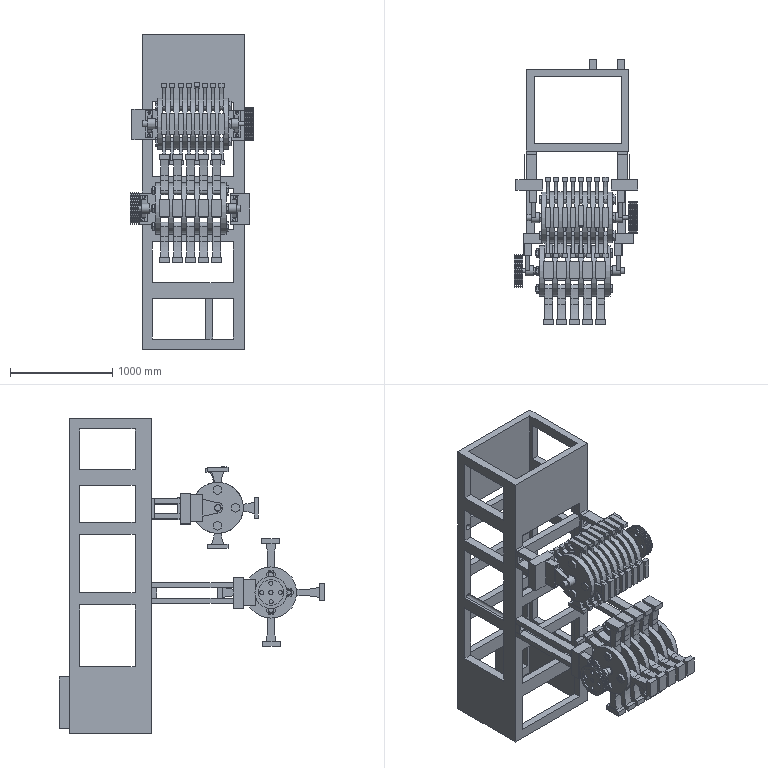Assembly | NX | mm | 108 component files | 114 solids | 1657 faces | box 1205 x 2593.88 x 3074.18 mm | volume 688918586 mm3 | plane 1034 | cylinder 559 | spline 32 | cone 32 | commonest cylinder face diameters 50 x213 1526.456 x80 580.798 x64 80 x60 60 x20 30 x16 500 x15 120 x13
Bill of materials:
unnamed part 1 | 11 |  | Thin flat circular disc with a central round bore that has a single keyway notch, and four smaller through-holes spaced evenly on a bolt circle.
unnamed part 2 | 4 |  | Rectangular mounting block with two through-holes near its ends, plus a tapered web arm that extends sideways to a cylindrical boss with a through-bore.
unnamed part 3 | 32 |  | Flat T-shaped plate: a rectangular bar head with an arm whose sides curve inward, ending in a rounded eye with a round through-hole.
unnamed part 4 | 8 |  | Hexagonal nut with a large central bore showing internal helical thread geometry; its height is small compared with its width across flats.
unnamed part 5 | 2 |  | Long open rectangular frame: two parallel bars joined by an end wall, attached to a wider rectangular end block that has two small through-holes.
unnamed part 6 | 2 |  | Long, slender, flat bar with rounded (semicircular) ends.
unnamed part 7 | 20 |  | T-shaped plate: a rectangular head block with a long arm whose sides curve slightly inward, ending in a rounded eye with a round through-hole.
unnamed part 8 | 2 |  | Multi-groove disc (pulley-like) with V-section grooves around its rim, a central bore with a keyway notch, four larger holes spaced evenly around it, and a shallow recess on the face.
unnamed part 9 | 2 |  | Stepped cylindrical shaft: a large central body with several smaller-diameter stepped sections at each end.
unnamed part 10 | 2 |  | Short open rectangular frame attached to a wide rectangular block that has two small holes on its face; the far end wall of the frame has a round hole.
unnamed part 11 | 2 |  | Thin flat circular disc with a plain central round hole and four smaller through-holes spaced evenly on a bolt circle.
unnamed part 12 | 8 |  | Long bolt-like part: a hexagonal head on a long cylindrical shank, with thread-like grooves on a short section at the far end.
unnamed part 13 | 8 |  | Thin flat circular ring with a rectangular cross-section and a large central opening
unnamed part 14 | 2 |  | Solid prism with a stadium-shaped (obround) cross-section: two flat parallel sides joined by semicircular ends, extruded to a uniform length
unnamed part 15 | 2 |  | Flat circular disc with one central through-hole and four smaller through-holes spaced evenly on a circle around it
unnamed part 16 | 1 |  | Tall, open, rectangular box-shaped frame of vertical posts, horizontal crossbars, and side panels with several rectangular openings; a closed panel section near the top and a protruding block near the bottom on one side
Mates:
1. concentric | main_shaft_key 1 | main_shaft 1
2. concentric | pulley_key 1 | main_shaft 1
3. concentric | outer_hammer_disc 2 | hammer_head_3 7
4. concentric | outer_hammer_disc 1 | hammer_head_3 3
5. concentric | rotor_disc 6 | hammer_head_3 7
6. concentric | rotor_disc 3 | hammer_head_3 11
7. concentric | rotor_disc 4 | hammer_head_3 15
8. concentric | rotor_disc 5 | hammer_head_3 22
9. concentric | rotor_disc 7 | hammer_head_3 23
10. concentric | rotor_disc 2 | hammer_head_3 26
11. concentric | rotor_disc 1 | hammer_head_3 32
12. concentric | pin_shaft_washer 4 | pin_nut 1
13. concentric | pin_shaft_washer 3 | pin_nut 2
14. concentric | pin_shaft_washer 2 | pin_nut 3
15. concentric | pin_shaft_washer 1 | pin_nut 4
16. concentric | pin_shaft_washer 4 | outer_hammer_disc 1
17. concentric | pin_shaft_washer 1 | outer_hammer_disc 1
18. concentric | pin_shaft_washer 2 | outer_hammer_disc 1
19. concentric | pin_shaft_washer 3 | outer_hammer_disc 1
20. concentric | pin_shaft_2 4 | outer_hammer_disc 2
21. concentric | pin_shaft_2 2 | outer_hammer_disc 2
22. concentric | pin_shaft_2 1 | outer_hammer_disc 2
23. concentric | pin_shaft_2 3 | outer_hammer_disc 2
24. concentric | shaft_2_assy 1 | outer_hammer_disc 2
25. concentric | upper_hammer 17 | outer_hammer_disc 2
26. concentric | rotor_disc 4 | upper_hammer 17
27. concentric | upper_hammer 20 | rotor_disc 4
28. concentric | upper_hammer 18 | outer_hammer_disc 2
29. concentric | upper_hammer 13 | outer_hammer_disc 2
30. concentric | upper_hammer 14 | outer_hammer_disc 2
31. concentric | upper_hammer 16 | rotor_disc 4
32. concentric | upper_hammer 15 | rotor_disc 4
33. concentric | upper_hammer 19 | rotor_disc 4
34. concentric | rotor_disc 3 | upper_hammer 20
35. concentric | upper_hammer 9 | rotor_disc 3
36. concentric | upper_hammer 12 | rotor_disc 3
37. concentric | upper_hammer 11 | rotor_disc 3
38. concentric | upper_hammer 10 | rotor_disc 3
39. concentric | rotor_disc 1 | upper_hammer 9
40. concentric | upper_hammer 7 | rotor_disc 1
41. concentric | upper_hammer 8 | rotor_disc 1
42. concentric | upper_hammer 6 | rotor_disc 1
43. concentric | upper_hammer 5 | rotor_disc 1
44. concentric | rotor_disc 2 | upper_hammer 7
45. concentric | upper_hammer 2 | rotor_disc 2
46. concentric | upper_hammer 1 | rotor_disc 2
47. concentric | upper_hammer 4 | rotor_disc 2
48. concentric | upper_hammer 3 | rotor_disc 2
49. concentric | outer_hammer_disc 1 | upper_hammer 2
50. concentric | pin_shaft_washer 4 | pin_nut 4
51. concentric | pin_shaft_washer 4 | outer_hammer_disc 1
52. concentric | pin_shaft_2 4 | outer_hammer_disc 2
53. concentric | pin_shaft_washer 3 | pin_nut 1
54. concentric | pin_shaft_washer 2 | pin_nut 3
55. concentric | pin_shaft_washer 1 | pin_nut 2
56. concentric | pin_shaft_washer 2 | outer_hammer_disc 1
57. concentric | pin_shaft_washer 3 | outer_hammer_disc 1
58. concentric | pin_shaft_washer 1 | outer_hammer_disc 1
59. concentric | pin_shaft_2 1 | outer_hammer_disc 2
60. concentric | pin_shaft_2 3 | outer_hammer_disc 2
61. concentric | pin_shaft_2 2 | outer_hammer_disc 2
62. concentric | shaft_2_assy 1 | outer_hammer_disc 2
63. concentric | lower_rotor 1 edge | bearing_housing 4 edge
64. concentric | lower_support_seat 2 | base 1
65. concentric | lower_support_seat 1 | base 1 edge
66. concentric | lower_support_seat 2 | base 1 edge
67. concentric | lower_support_seat 1 arc | base 1 edge
68. concentric | lower_support_seat 2 arc | base 1 edge
69. concentric | large_pulley 2 arc | lower_rotor 1 edge
70. concentric | upper_support_seat 2 arc | base 1 edge
71. concentric | bearing_housing 1 arc | upper_rotor 1 edge
72. concentric | bearing_housing 1 edge | upper_support_seat 2 arc
73. concentric | upper_support_seat 1 arc | base 1 edge
74. concentric | bearing_housing 2 edge | upper_support_seat 1 arc
75. concentric | large_pulley 1 edge | upper_rotor 1 edge